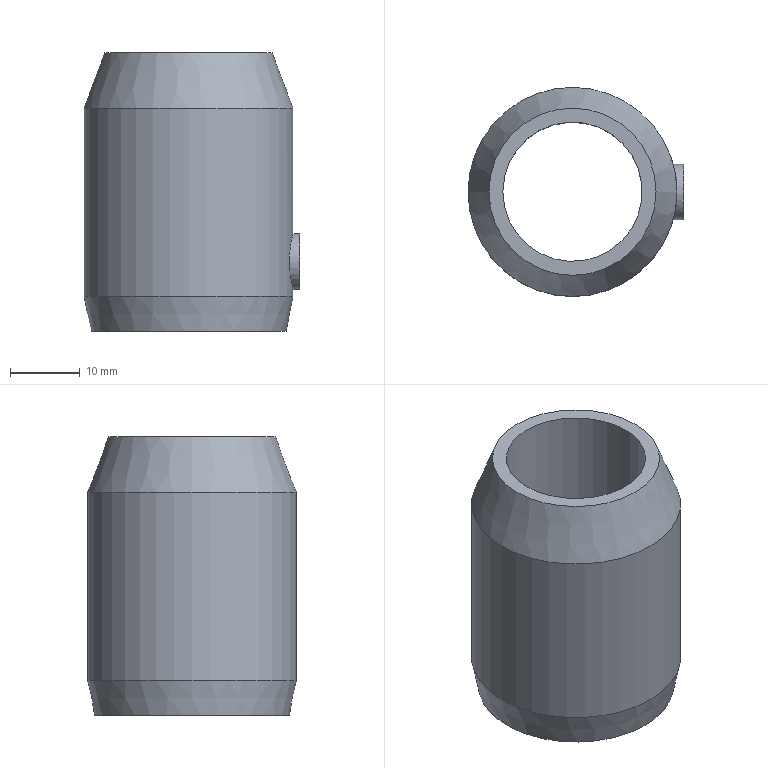Component | NX | LOCK_SLEEVE | 1 solid | 11 faces | volume 10875 mm3 | cylinder 5 | plane 4 | cone 2 | commonest cylinder face diameters 30 x1 20 x1 25 x1 8 x1 5 x1